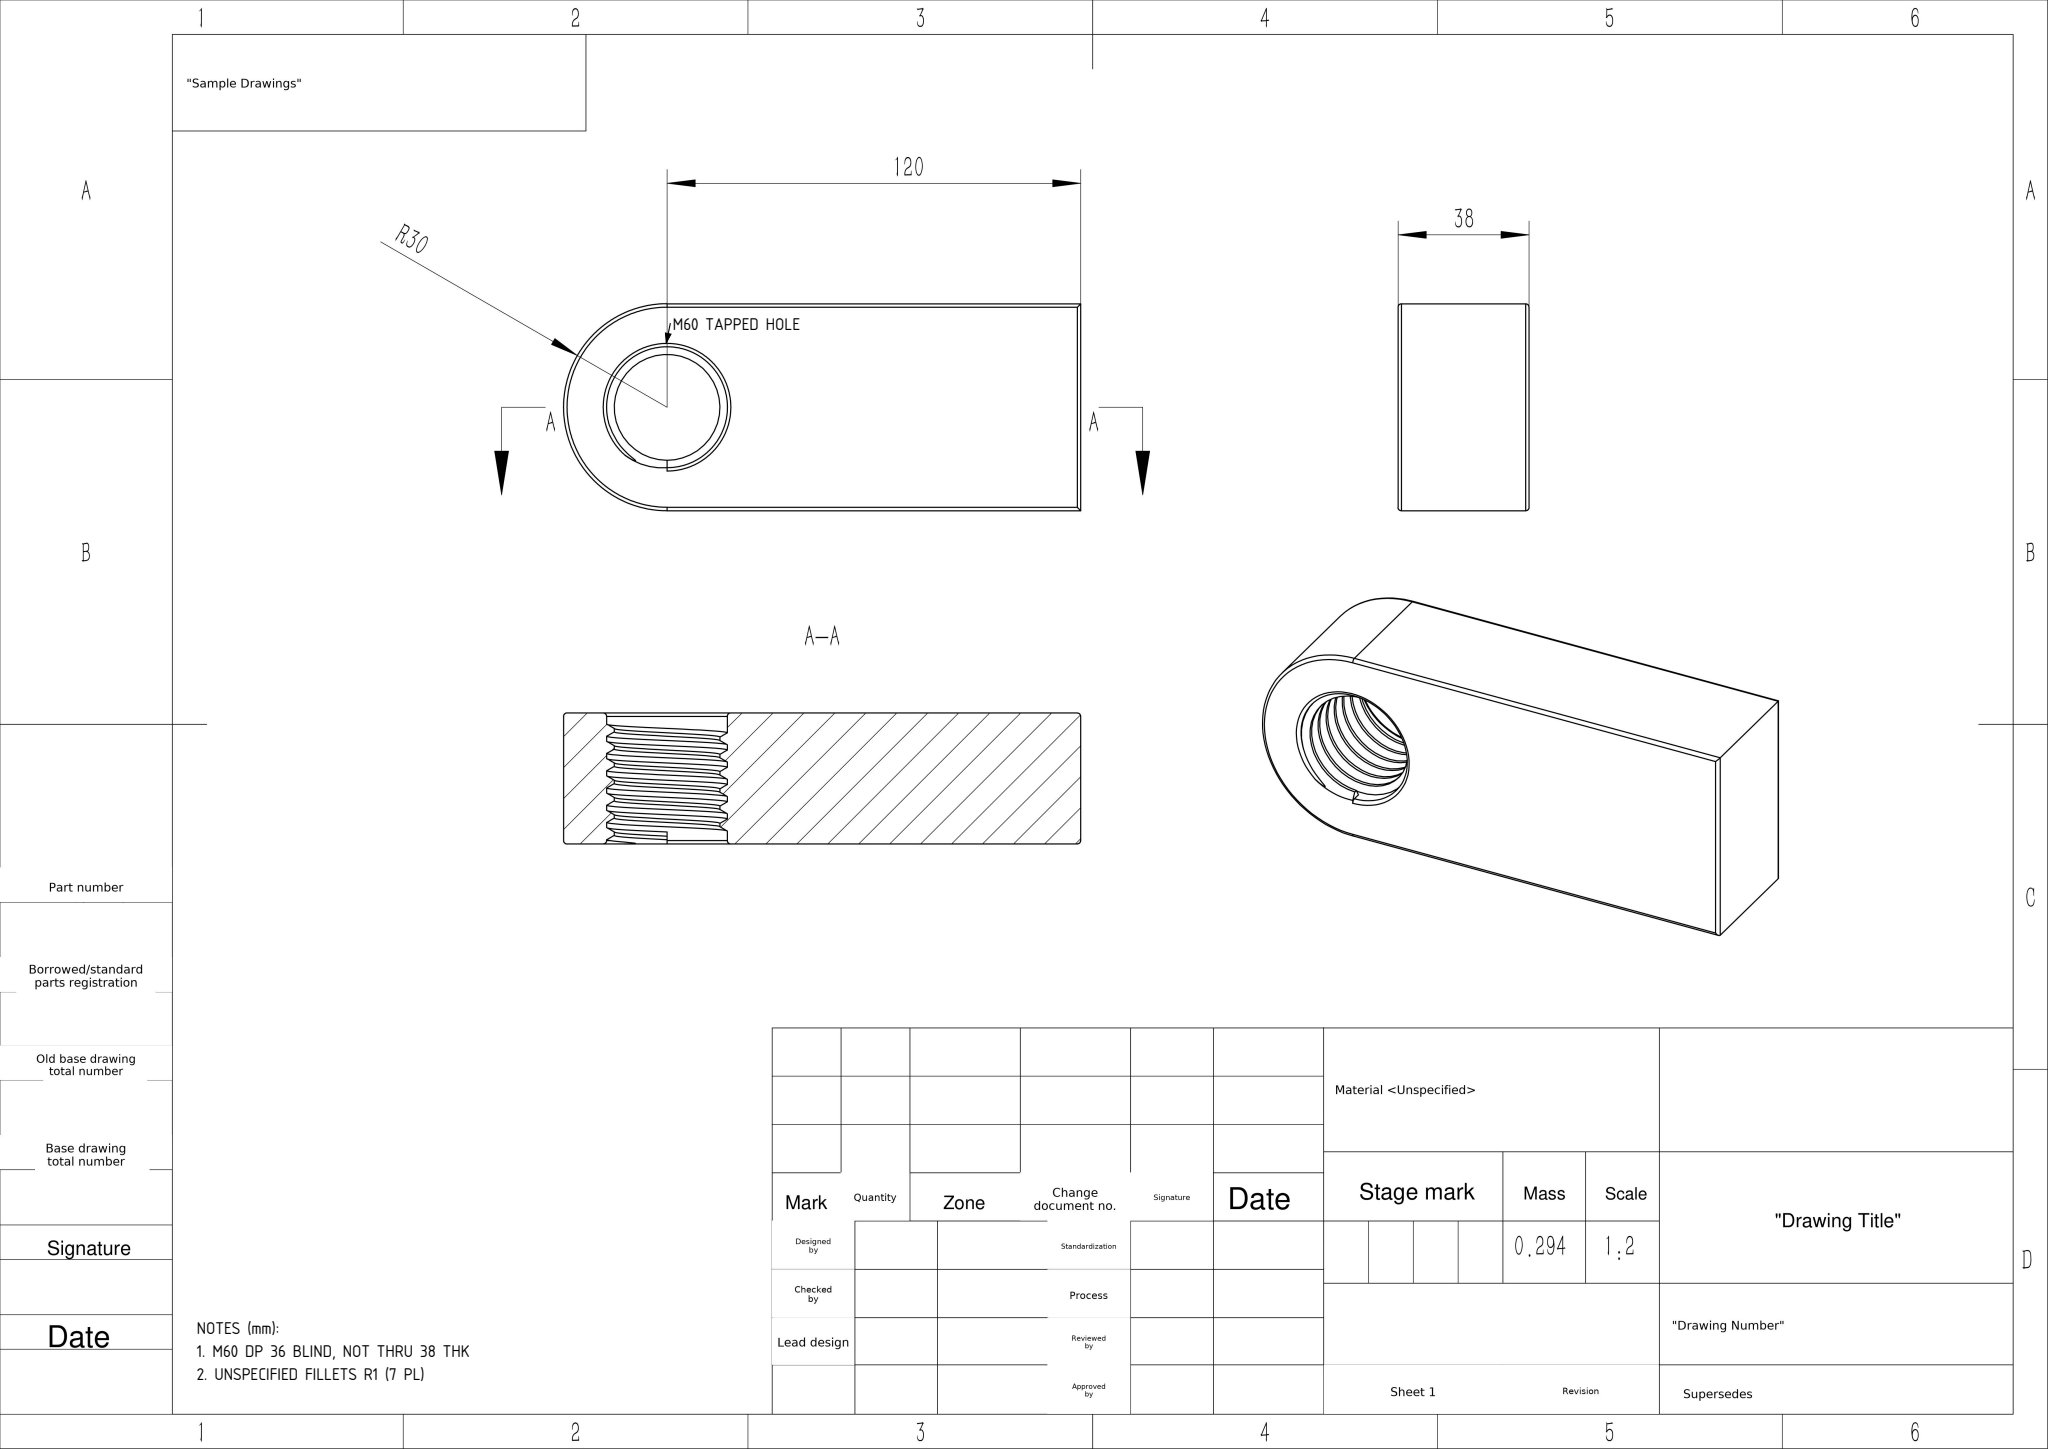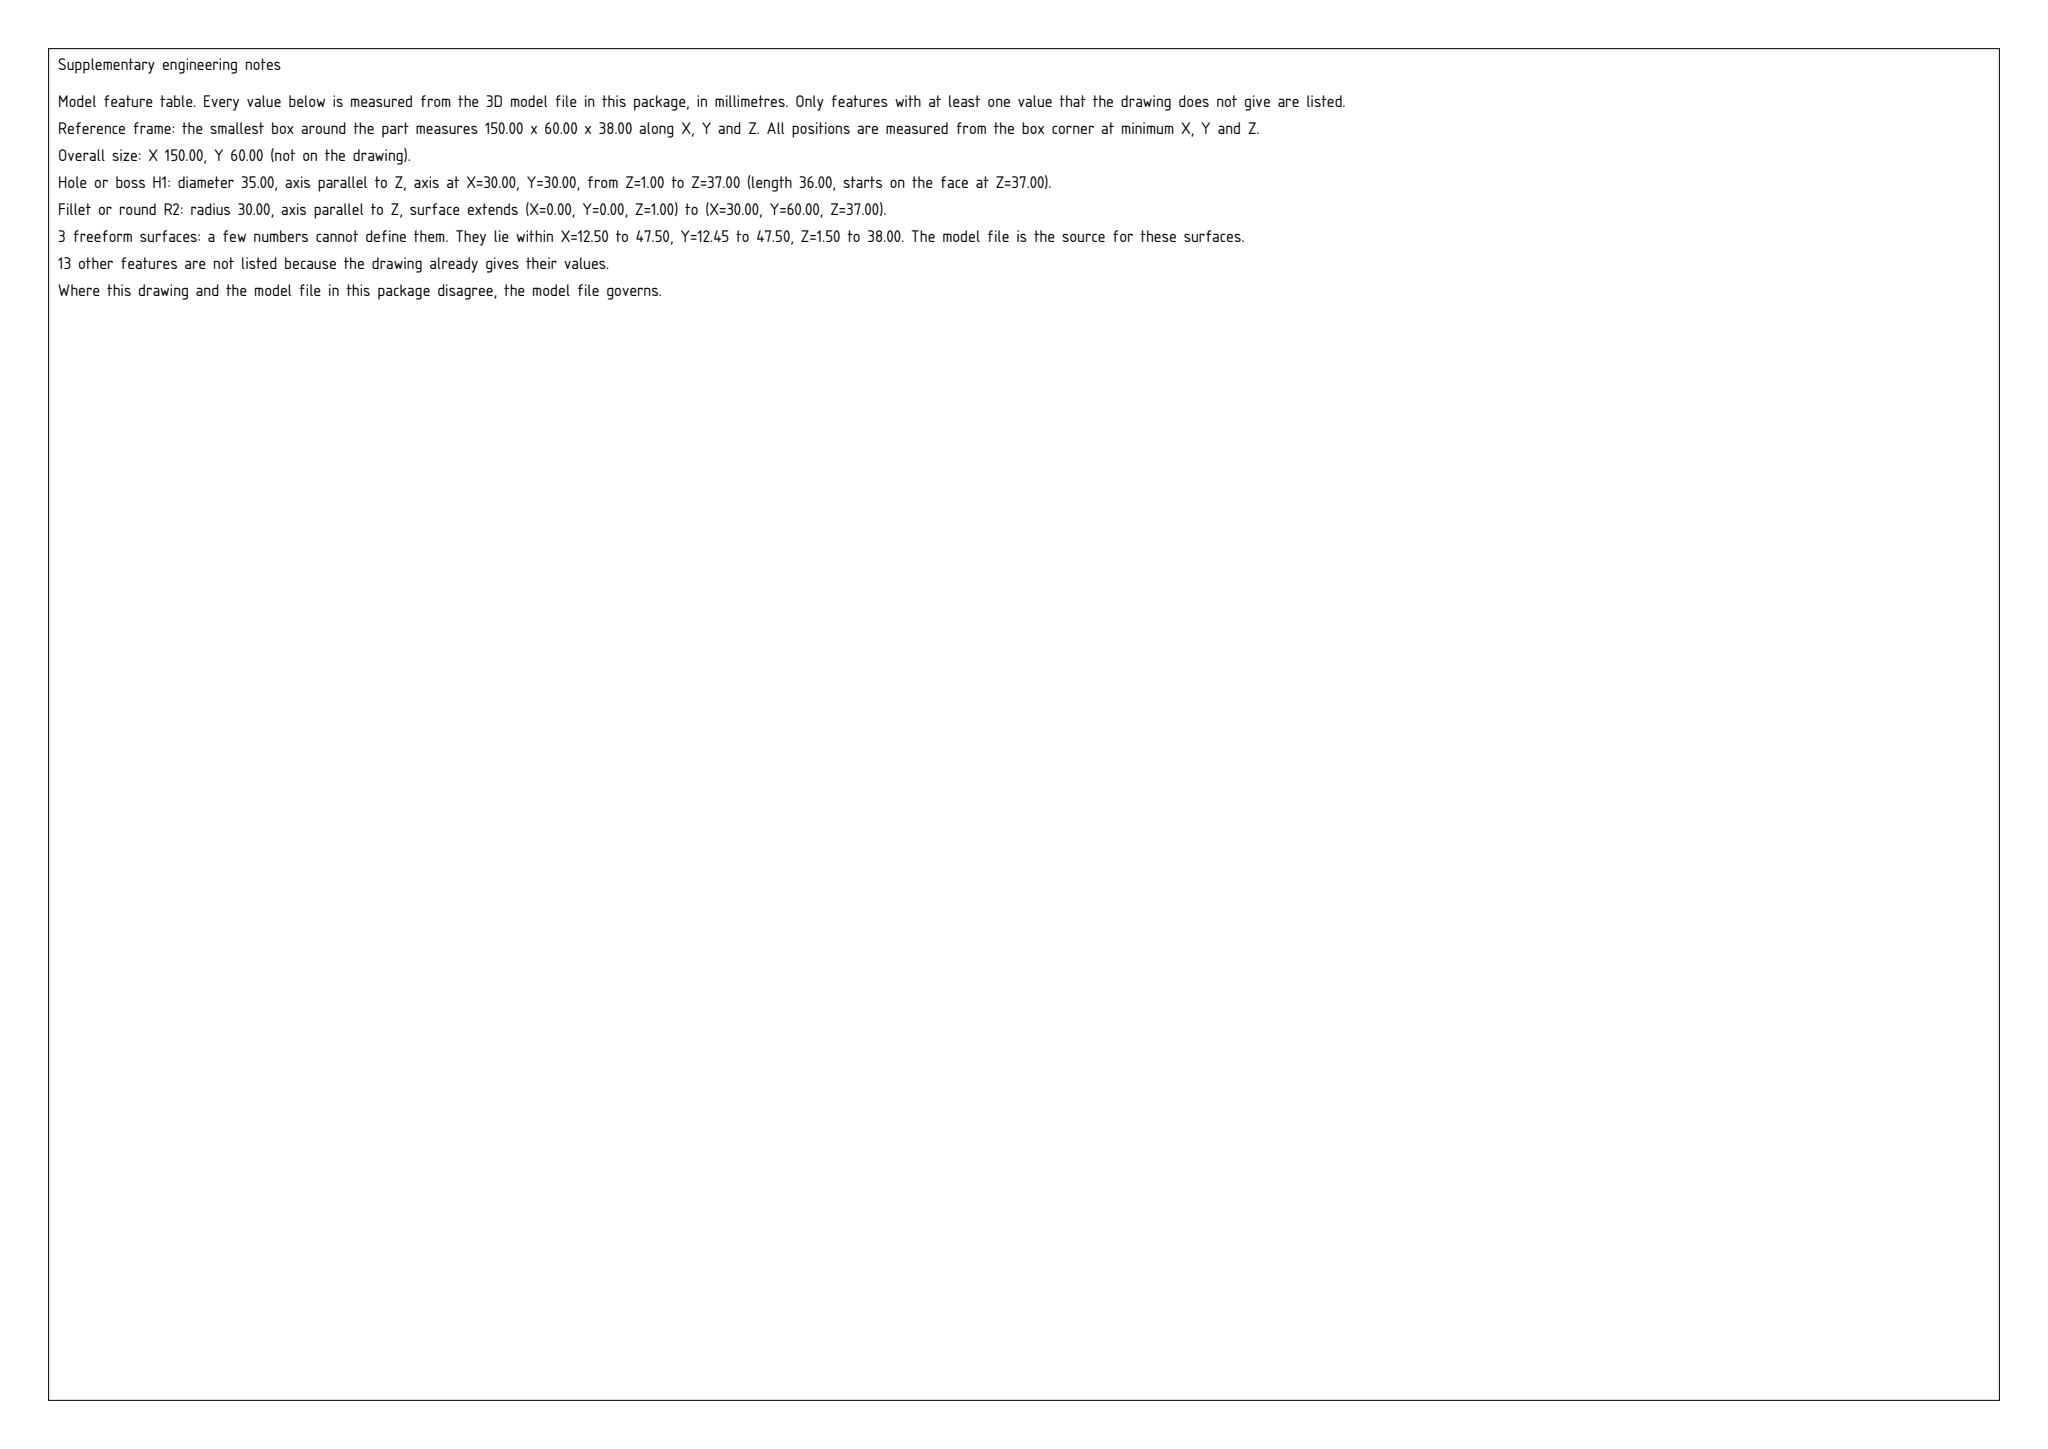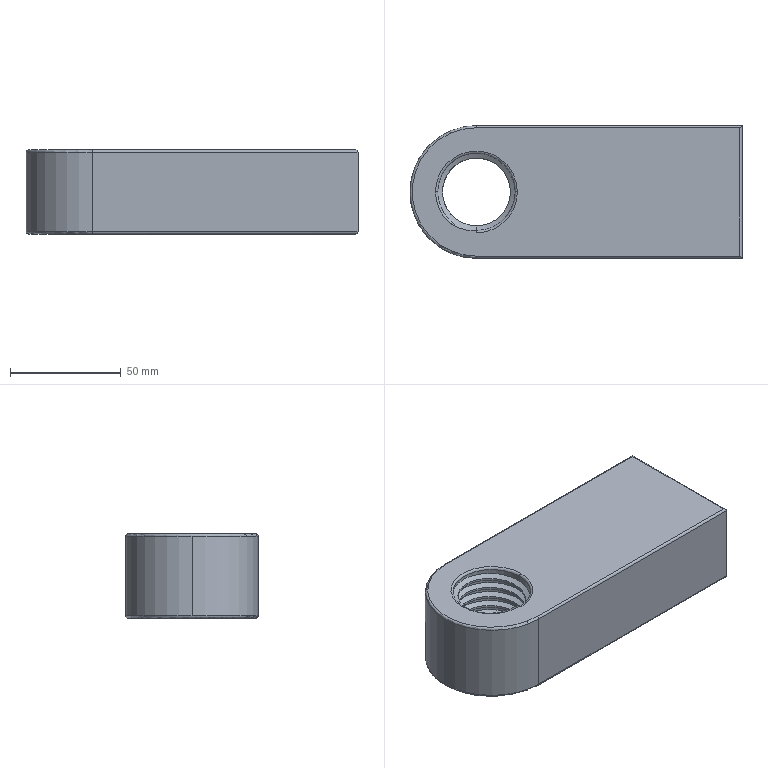Part | SolidWorks | mm | 1 solid | 40 faces | box 150 x 60 x 38 mm | volume 293893 mm3 | cylinder 23 | torus 7 | plane 7 | spline 3 | commonest cylinder face diameters 35 x15 2 x6 60 x2
Drawing notes:
TAPPED HOLE M60, CL AT R30 CTR (TOP VIEW & A-A) | from the solid: Ø60 z-axis cylinder at (32.47,32.47), thread profile rings Ø35
M60 DP 36 BLIND, NOT THRU 38 THK | from the solid: Ø60 bore length 36.0 vs z-planes 0.0 and 38.0
UNSPECIFIED FILLETS R1 (7 PL) | from the solid: fillet_radii: [[1.0, 7]]